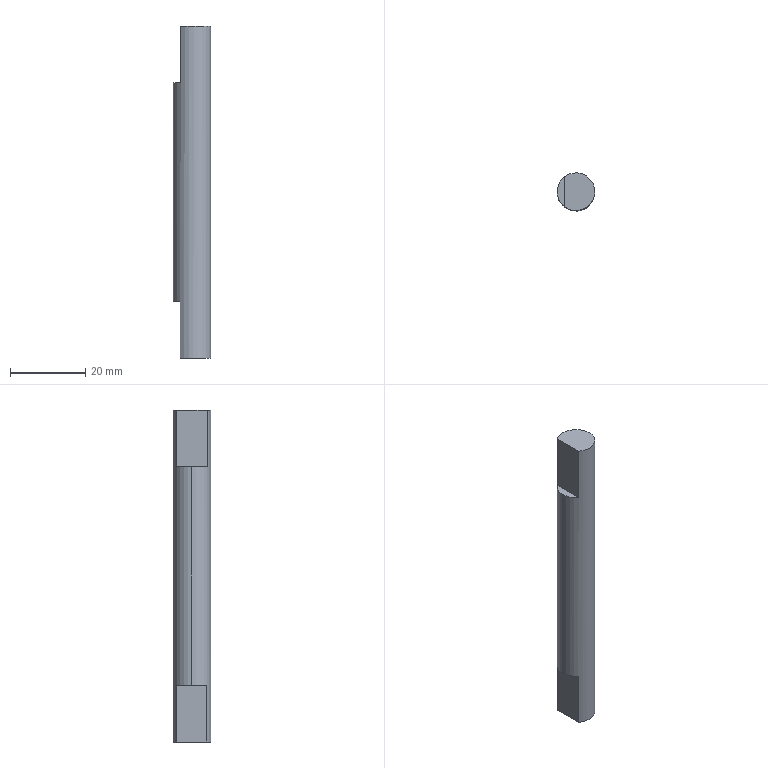Component | SolidWorks | --MA18S2004110mmSolderingIron-1 | 1 solid | 9 faces | box 10 x 10 x 88 mm | volume 6576 mm3 | plane 7 | cylinder 2 | commonest cylinder face diameters 10 x2
build123d program:
from build123d import *

# Parameters (mm, degrees)
SKETCH1_R           = 5
BOSS_EXTRUDE1_DEPTH = 88
SKETCH2_W           = 4.184
SKETCH2_H           = 10.917
CUT_EXTRUDE1_DEPTH  = 15
SKETCH3_W           = 3.437
SKETCH3_H           = 7.918
CUT_EXTRUDE2_DEPTH  = 15


with BuildPart() as part:
    # Sketch1 → Boss-Extrude1 (new body)
    with BuildSketch(Plane.XY):
        Circle(SKETCH1_R)
    extrude(amount=BOSS_EXTRUDE1_DEPTH)

    # Sketch2 → Cut-Extrude1 (cut)
    with BuildSketch(Plane.XY.offset(88)):
        with Locations((-5.092, 0.1202)):
            Rectangle(SKETCH2_W, SKETCH2_H)
    extrude(amount=-CUT_EXTRUDE1_DEPTH, mode=Mode.SUBTRACT)

    # Sketch3 → Cut-Extrude2 (cut)
    with BuildSketch(Plane(origin=(0, 0, 0), x_dir=(-1, 0, 0), z_dir=(0, 0, -1))):
        with Locations((4.719, 0.0487)):
            Rectangle(SKETCH3_W, SKETCH3_H)
    extrude(amount=-CUT_EXTRUDE2_DEPTH, mode=Mode.SUBTRACT)


solid = part.part

# Placed as in the assembly
solid = solid.moved(Location((12.044, 38.699, -10), (0, 0, 0)))
STEP:
#1=COLOUR_RGB('',0.7922,0.8196,0.9333);
#2=FILL_AREA_STYLE_COLOUR('',#1);
#3=FILL_AREA_STYLE('',(#2));
#4=SURFACE_STYLE_FILL_AREA(#3);
#5=SURFACE_SIDE_STYLE('',(#4));
#6=SURFACE_STYLE_USAGE(.BOTH.,#5);
#7=PRESENTATION_STYLE_ASSIGNMENT((#6));
#8=CARTESIAN_POINT('',(0.671,1.523,3.071));
#9=VERTEX_POINT('',#8);
#10=CARTESIAN_POINT('',(0.3563,1.681,3.071));
#11=VERTEX_POINT('',#10);
#12=CARTESIAN_POINT('',(0.4742,1.524,3.071));
#13=DIRECTION('',(0.,0.,1.));
#14=DIRECTION('',(1.,-0.001494,0.));
#15=AXIS2_PLACEMENT_3D('',#12,#13,#14);
#16=CIRCLE('',#15,0.1969);
#17=EDGE_CURVE('',#9,#11,#16,.T.);
#18=ORIENTED_EDGE('',*,*,#17,.F.);
#19=CARTESIAN_POINT('',(0.671,1.523,-0.3937));
#20=VERTEX_POINT('',#19);
#21=CARTESIAN_POINT('',(0.671,1.523,3.071));
#22=DIRECTION('',(0.,0.,-1.));
#23=VECTOR('',#22,39.37);
#24=LINE('',#21,#23);
#25=EDGE_CURVE('',#9,#20,#24,.T.);
#26=ORIENTED_EDGE('',*,*,#25,.T.);
#27=CARTESIAN_POINT('',(0.3563,1.681,-0.3937));
#28=VERTEX_POINT('',#27);
#29=CARTESIAN_POINT('',(0.4742,1.524,-0.3937));
#30=DIRECTION('',(0.,0.,1.));
#31=DIRECTION('',(1.,-0.001494,0.));
#32=AXIS2_PLACEMENT_3D('',#29,#30,#31);
#33=CIRCLE('',#32,0.1969);
#34=EDGE_CURVE('',#20,#28,#33,.T.);
#35=ORIENTED_EDGE('',*,*,#34,.T.);
#36=CARTESIAN_POINT('',(0.3563,1.681,0.1969));
#37=VERTEX_POINT('',#36);
#38=CARTESIAN_POINT('',(0.3563,1.681,3.071));
#39=DIRECTION('',(0.,0.,1.));
#40=VECTOR('',#39,39.37);
#41=LINE('',#38,#40);
#42=EDGE_CURVE('',#28,#37,#41,.T.);
#43=ORIENTED_EDGE('',*,*,#42,.T.);
#44=CARTESIAN_POINT('',(0.2773,1.524,0.1969));
#45=VERTEX_POINT('',#44);
#46=CARTESIAN_POINT('',(0.4742,1.524,0.1969));
#47=DIRECTION('',(0.,0.,-1.));
#48=DIRECTION('',(-1.,0.001494,0.));
#49=AXIS2_PLACEMENT_3D('',#46,#47,#48);
#50=CIRCLE('',#49,0.1969);
#51=EDGE_CURVE('',#45,#37,#50,.T.);
#52=ORIENTED_EDGE('',*,*,#51,.F.);
#53=CARTESIAN_POINT('',(0.2773,1.524,2.48));
#54=VERTEX_POINT('',#53);
#55=CARTESIAN_POINT('',(0.2773,1.524,3.071));
#56=DIRECTION('',(0.,0.,-1.));
#57=VECTOR('',#56,39.37);
#58=LINE('',#55,#57);
#59=EDGE_CURVE('',#54,#45,#58,.T.);
#60=ORIENTED_EDGE('',*,*,#59,.F.);
#61=CARTESIAN_POINT('',(0.3563,1.681,2.48));
#62=VERTEX_POINT('',#61);
#63=CARTESIAN_POINT('',(0.4742,1.524,2.48));
#64=DIRECTION('',(0.,0.,1.));
#65=DIRECTION('',(1.,-0.001494,0.));
#66=AXIS2_PLACEMENT_3D('',#63,#64,#65);
#67=CIRCLE('',#66,0.1969);
#68=EDGE_CURVE('',#62,#54,#67,.T.);
#69=ORIENTED_EDGE('',*,*,#68,.F.);
#70=CARTESIAN_POINT('',(0.3563,1.681,3.071));
#71=DIRECTION('',(0.,0.,1.));
#72=VECTOR('',#71,39.37);
#73=LINE('',#70,#72);
#74=EDGE_CURVE('',#62,#11,#73,.T.);
#75=ORIENTED_EDGE('',*,*,#74,.T.);
#76=EDGE_LOOP('',(#18,#26,#35,#43,#52,#60,#69,#75));
#77=FACE_OUTER_BOUND('',#76,.T.);
#78=CARTESIAN_POINT('',(0.4742,1.524,3.071));
#79=DIRECTION('',(0.,0.,-1.));
#80=DIRECTION('',(-1.,0.001494,0.));
#81=AXIS2_PLACEMENT_3D('',#78,#79,#80);
#82=CYLINDRICAL_SURFACE('',#81,0.1969);
#83=ADVANCED_FACE('',(#77),#82,.T.);
#84=ORIENTED_EDGE('',*,*,#25,.F.);
#85=CARTESIAN_POINT('',(0.3558,1.366,3.071));
#86=VERTEX_POINT('',#85);
#87=CARTESIAN_POINT('',(0.4742,1.524,3.071));
#88=DIRECTION('',(0.,0.,1.));
#89=DIRECTION('',(1.,-0.001494,0.));
#90=AXIS2_PLACEMENT_3D('',#87,#88,#89);
#91=CIRCLE('',#90,0.1969);
#92=EDGE_CURVE('',#86,#9,#91,.T.);
#93=ORIENTED_EDGE('',*,*,#92,.F.);
#94=CARTESIAN_POINT('',(0.3558,1.366,2.48));
#95=VERTEX_POINT('',#94);
#96=CARTESIAN_POINT('',(0.3558,1.366,3.071));
#97=DIRECTION('',(0.,0.,-1.));
#98=VECTOR('',#97,39.37);
#99=LINE('',#96,#98);
#100=EDGE_CURVE('',#86,#95,#99,.T.);
#101=ORIENTED_EDGE('',*,*,#100,.T.);
#102=CARTESIAN_POINT('',(0.4742,1.524,2.48));
#103=DIRECTION('',(0.,0.,1.));
#104=DIRECTION('',(1.,-0.001494,0.));
#105=AXIS2_PLACEMENT_3D('',#102,#103,#104);
#106=CIRCLE('',#105,0.1969);
#107=EDGE_CURVE('',#54,#95,#106,.T.);
#108=ORIENTED_EDGE('',*,*,#107,.F.);
#109=ORIENTED_EDGE('',*,*,#59,.T.);
#110=CARTESIAN_POINT('',(0.3513,1.37,0.1969));
#111=VERTEX_POINT('',#110);
#112=CARTESIAN_POINT('',(0.4742,1.524,0.1969));
#113=DIRECTION('',(0.,0.,-1.));
#114=DIRECTION('',(-1.,0.001494,0.));
#115=AXIS2_PLACEMENT_3D('',#112,#113,#114);
#116=CIRCLE('',#115,0.1969);
#117=EDGE_CURVE('',#111,#45,#116,.T.);
#118=ORIENTED_EDGE('',*,*,#117,.F.);
#119=CARTESIAN_POINT('',(0.3513,1.37,-0.3937));
#120=VERTEX_POINT('',#119);
#121=CARTESIAN_POINT('',(0.3513,1.37,3.071));
#122=DIRECTION('',(0.,0.,-1.));
#123=VECTOR('',#122,39.37);
#124=LINE('',#121,#123);
#125=EDGE_CURVE('',#111,#120,#124,.T.);
#126=ORIENTED_EDGE('',*,*,#125,.T.);
#127=CARTESIAN_POINT('',(0.4742,1.524,-0.3937));
#128=DIRECTION('',(0.,0.,1.));
#129=DIRECTION('',(1.,-0.001494,0.));
#130=AXIS2_PLACEMENT_3D('',#127,#128,#129);
#131=CIRCLE('',#130,0.1969);
#132=EDGE_CURVE('',#120,#20,#131,.T.);
#133=ORIENTED_EDGE('',*,*,#132,.T.);
#134=EDGE_LOOP('',(#84,#93,#101,#108,#109,#118,#126,#133));
#135=FACE_OUTER_BOUND('',#134,.T.);
#136=CARTESIAN_POINT('',(0.4742,1.524,3.071));
#137=DIRECTION('',(0.,0.,-1.));
#138=DIRECTION('',(-1.,0.001494,0.));
#139=AXIS2_PLACEMENT_3D('',#136,#137,#138);
#140=CYLINDRICAL_SURFACE('',#139,0.1969);
#141=ADVANCED_FACE('',(#135),#140,.T.);
#142=CARTESIAN_POINT('',(0.3561,1.524,3.071));
#143=DIRECTION('',(0.001494,1.,0.));
#144=VECTOR('',#143,39.37);
#145=LINE('',#142,#144);
#146=EDGE_CURVE('',#86,#11,#145,.T.);
#147=ORIENTED_EDGE('',*,*,#146,.F.);
#148=ORIENTED_EDGE('',*,*,#92,.T.);
#149=ORIENTED_EDGE('',*,*,#17,.T.);
#150=EDGE_LOOP('',(#147,#148,#149));
#151=FACE_OUTER_BOUND('',#150,.T.);
#152=CARTESIAN_POINT('',(0.4742,1.524,3.071));
#153=DIRECTION('',(0.,0.,1.));
#154=DIRECTION('',(1.,-0.001494,0.));
#155=AXIS2_PLACEMENT_3D('',#152,#153,#154);
#156=PLANE('',#155);
#157=ADVANCED_FACE('',(#151),#156,.T.);
#158=CARTESIAN_POINT('',(0.3558,1.37,-0.3937));
#159=VERTEX_POINT('',#158);
#160=CARTESIAN_POINT('',(0.3558,1.37,-0.3937));
#161=DIRECTION('',(-1.,0.001494,0.));
#162=VECTOR('',#161,39.37);
#163=LINE('',#160,#162);
#164=EDGE_CURVE('',#159,#120,#163,.T.);
#165=ORIENTED_EDGE('',*,*,#164,.F.);
#166=CARTESIAN_POINT('',(0.3561,1.524,-0.3937));
#167=DIRECTION('',(0.001494,1.,0.));
#168=VECTOR('',#167,39.37);
#169=LINE('',#166,#168);
#170=EDGE_CURVE('',#159,#28,#169,.T.);
#171=ORIENTED_EDGE('',*,*,#170,.T.);
#172=ORIENTED_EDGE('',*,*,#34,.F.);
#173=ORIENTED_EDGE('',*,*,#132,.F.);
#174=EDGE_LOOP('',(#165,#171,#172,#173));
#175=FACE_OUTER_BOUND('',#174,.T.);
#176=CARTESIAN_POINT('',(0.4742,1.524,-0.3937));
#177=DIRECTION('',(0.,0.,1.));
#178=DIRECTION('',(1.,-0.001494,0.));
#179=AXIS2_PLACEMENT_3D('',#176,#177,#178);
#180=PLANE('',#179);
#181=ADVANCED_FACE('',(#175),#180,.F.);
#182=ORIENTED_EDGE('',*,*,#68,.T.);
#183=ORIENTED_EDGE('',*,*,#107,.T.);
#184=CARTESIAN_POINT('',(0.3564,1.743,2.48));
#185=DIRECTION('',(0.001494,1.,0.));
#186=VECTOR('',#185,39.37);
#187=LINE('',#184,#186);
#188=EDGE_CURVE('',#95,#62,#187,.T.);
#189=ORIENTED_EDGE('',*,*,#188,.T.);
#190=EDGE_LOOP('',(#182,#183,#189));
#191=FACE_OUTER_BOUND('',#190,.T.);
#192=CARTESIAN_POINT('',(0.191,1.314,2.48));
#193=DIRECTION('',(0.,0.,1.));
#194=DIRECTION('',(1.,-0.001494,0.));
#195=AXIS2_PLACEMENT_3D('',#192,#193,#194);
#196=PLANE('',#195);
#197=ADVANCED_FACE('',(#191),#196,.T.);
#198=ORIENTED_EDGE('',*,*,#146,.T.);
#199=ORIENTED_EDGE('',*,*,#74,.F.);
#200=ORIENTED_EDGE('',*,*,#188,.F.);
#201=ORIENTED_EDGE('',*,*,#100,.F.);
#202=EDGE_LOOP('',(#198,#199,#200,#201));
#203=FACE_OUTER_BOUND('',#202,.T.);
#204=CARTESIAN_POINT('',(0.3564,1.743,2.48));
#205=DIRECTION('',(1.,-0.001494,0.));
#206=DIRECTION('',(0.001494,1.,0.));
#207=AXIS2_PLACEMENT_3D('',#204,#205,#206);
#208=PLANE('',#207);
#209=ADVANCED_FACE('',(#203),#208,.F.);
#210=ORIENTED_EDGE('',*,*,#117,.T.);
#211=ORIENTED_EDGE('',*,*,#51,.T.);
#212=CARTESIAN_POINT('',(0.3558,1.37,0.1969));
#213=VERTEX_POINT('',#212);
#214=CARTESIAN_POINT('',(0.3563,1.682,0.1969));
#215=DIRECTION('',(-0.001494,-1.,0.));
#216=VECTOR('',#215,39.37);
#217=LINE('',#214,#216);
#218=EDGE_CURVE('',#37,#213,#217,.T.);
#219=ORIENTED_EDGE('',*,*,#218,.T.);
#220=CARTESIAN_POINT('',(0.3558,1.37,0.1969));
#221=DIRECTION('',(-1.,0.001494,0.));
#222=VECTOR('',#221,39.37);
#223=LINE('',#220,#222);
#224=EDGE_CURVE('',#213,#111,#223,.T.);
#225=ORIENTED_EDGE('',*,*,#224,.T.);
#226=EDGE_LOOP('',(#210,#211,#219,#225));
#227=FACE_OUTER_BOUND('',#226,.T.);
#228=CARTESIAN_POINT('',(0.3558,1.37,0.1969));
#229=DIRECTION('',(0.,0.,-1.));
#230=DIRECTION('',(-1.,0.001494,0.));
#231=AXIS2_PLACEMENT_3D('',#228,#229,#230);
#232=PLANE('',#231);
#233=ADVANCED_FACE('',(#227),#232,.T.);
#234=ORIENTED_EDGE('',*,*,#170,.F.);
#235=CARTESIAN_POINT('',(0.3558,1.37,0.1969));
#236=DIRECTION('',(0.,0.,-1.));
#237=VECTOR('',#236,39.37);
#238=LINE('',#235,#237);
#239=EDGE_CURVE('',#213,#159,#238,.T.);
#240=ORIENTED_EDGE('',*,*,#239,.F.);
#241=ORIENTED_EDGE('',*,*,#218,.F.);
#242=ORIENTED_EDGE('',*,*,#42,.F.);
#243=EDGE_LOOP('',(#234,#240,#241,#242));
#244=FACE_OUTER_BOUND('',#243,.T.);
#245=CARTESIAN_POINT('',(0.3563,1.682,0.1969));
#246=DIRECTION('',(1.,-0.001494,0.));
#247=DIRECTION('',(0.001494,1.,0.));
#248=AXIS2_PLACEMENT_3D('',#245,#246,#247);
#249=PLANE('',#248);
#250=ADVANCED_FACE('',(#244),#249,.F.);
#251=ORIENTED_EDGE('',*,*,#224,.F.);
#252=ORIENTED_EDGE('',*,*,#239,.T.);
#253=ORIENTED_EDGE('',*,*,#164,.T.);
#254=ORIENTED_EDGE('',*,*,#125,.F.);
#255=EDGE_LOOP('',(#251,#252,#253,#254));
#256=FACE_OUTER_BOUND('',#255,.T.);
#257=CARTESIAN_POINT('',(0.3558,1.37,0.1969));
#258=DIRECTION('',(-0.001494,-1.,0.));
#259=DIRECTION('',(0.,0.,-1.));
#260=AXIS2_PLACEMENT_3D('',#257,#258,#259);
#261=PLANE('',#260);
#262=ADVANCED_FACE('',(#256),#261,.F.);
#263=CLOSED_SHELL('',(#83,#141,#157,#181,#197,#209,#233,#250,#262));
#264=MANIFOLD_SOLID_BREP('',#263);
#265=STYLED_ITEM('',(#7),#264);
#266=(LENGTH_UNIT()NAMED_UNIT(*)SI_UNIT($,.METRE.));
#267=LENGTH_MEASURE_WITH_UNIT(LENGTH_MEASURE(0.0254),#266);
#268=DIMENSIONAL_EXPONENTS(1.,0.,0.,0.,0.,0.,0.);
#269=(CONVERSION_BASED_UNIT('',#267)LENGTH_UNIT()NAMED_UNIT(#268));
#270=UNCERTAINTY_MEASURE_WITH_UNIT(LENGTH_MEASURE(0.00001),#269,'','');
#271=(NAMED_UNIT(*)PLANE_ANGLE_UNIT()SI_UNIT($,.RADIAN.));
#272=(NAMED_UNIT(*)SI_UNIT($,.STERADIAN.)SOLID_ANGLE_UNIT());
#273=(GEOMETRIC_REPRESENTATION_CONTEXT(3)GLOBAL_UNCERTAINTY_ASSIGNED_CONTEXT((#270))GLOBAL_UNIT_ASSIGNED_CONTEXT((#269,#271,#272))REPRESENTATION_CONTEXT('',''));
#274=MECHANICAL_DESIGN_GEOMETRIC_PRESENTATION_REPRESENTATION('',(#265),#273);
#275=PRESENTATION_LAYER_ASSIGNMENT('','',(#265));
#276=CARTESIAN_POINT('',(0.,0.,0.));
#277=DIRECTION('',(0.,0.,1.));
#278=DIRECTION('',(1.,0.,0.));
#279=AXIS2_PLACEMENT_3D('',#276,#277,#278);
#280=(LENGTH_UNIT()NAMED_UNIT(*)SI_UNIT($,.METRE.));
#281=LENGTH_MEASURE_WITH_UNIT(LENGTH_MEASURE(0.0254),#280);
#282=DIMENSIONAL_EXPONENTS(1.,0.,0.,0.,0.,0.,0.);
#283=(CONVERSION_BASED_UNIT('',#281)LENGTH_UNIT()NAMED_UNIT(#282));
#284=UNCERTAINTY_MEASURE_WITH_UNIT(LENGTH_MEASURE(0.00001),#283,'','');
#285=(NAMED_UNIT(*)PLANE_ANGLE_UNIT()SI_UNIT($,.RADIAN.));
#286=(NAMED_UNIT(*)SI_UNIT($,.STERADIAN.)SOLID_ANGLE_UNIT());
#287=(GEOMETRIC_REPRESENTATION_CONTEXT(3)GLOBAL_UNCERTAINTY_ASSIGNED_CONTEXT((#284))GLOBAL_UNIT_ASSIGNED_CONTEXT((#283,#285,#286))REPRESENTATION_CONTEXT('',''));
#288=ADVANCED_BREP_SHAPE_REPRESENTATION('',(#264,#279),#287);